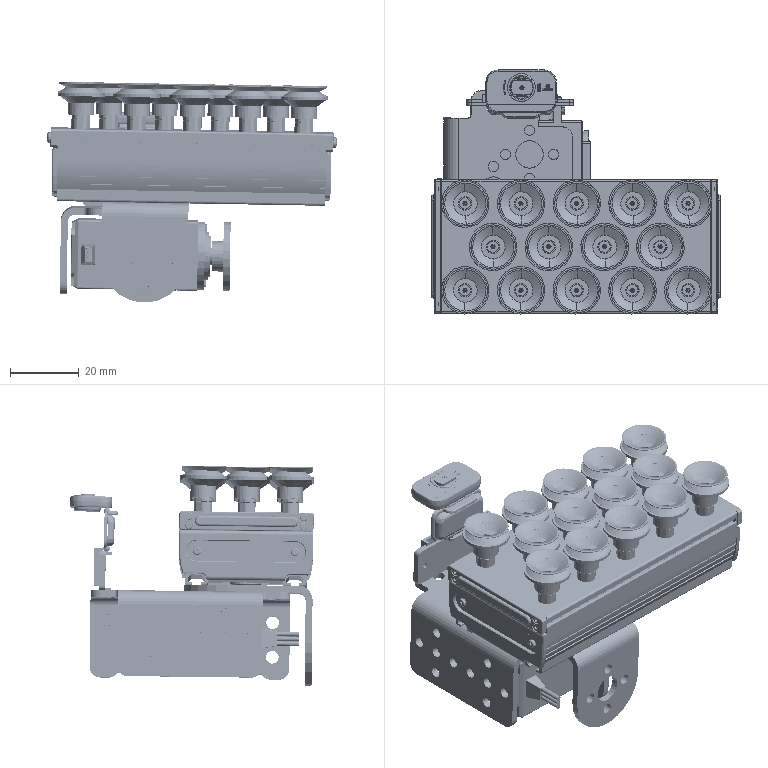Assembly | SolidWorks | mm | 78 component files | 81 solids | 4915 faces | box 84.02 x 70.93 x 64.22 mm | volume 84941 mm3 | cylinder 2079 | plane 1683 | cone 802 | spline 291 | torus 36 | sphere 24 | commonest cylinder face diameters 1.623 x328 2.074 x328 5.4 x168 1.8 x90 3 x78 5.8 x75 1.2 x74 3.3 x56
Bill of materials:
01-Profile | 1 |  | Long, constant-section, open-bottom channel-shaped profile with a flat top plate pierced by a staggered grid of holes, plus longitudinal grooves and slots along the side walls and foot features.
02-TopCoverPlate | 1 |  | Thin, flat rectangular plate with a U-shaped open slot coming in from one short end.
03-EndPlate | 2 |  | Thin plate, roughly rectangular, with a raised or recessed obround pad on one face, two small through holes, rounded edges and a stepped tab on one long edge.
04-SealingPlate | 2 |  | Long, narrow rectangular bar with chamfered corners, a long raised obround rib along one face, and two pairs of holes at the ends.
05-M4Screw | 8 |  | Socket-head screw-like shape: a cylindrical head with a hex socket and a smooth cylindrical shank with a chamfered tip.
06-M4PhillipsScrew | 4 |  | Pan- or cheese-head screw-like shape with a cross-shaped recess in the head and a smooth cylindrical shank with a chamfered tip.
07-Busbar | 1 |  | Rectangular block with chamfered corners and a stepped cylindrical spigot sticking out of one face near one end.
08-SoftRubberSuctionCup | 14 |  | Rotationally symmetric part with a cup shape: a conical inner bowl, two stacked flared lips or flanges, and a cylindrical stem with a small central through hole.
09-SuctionCupConnector | 14 |  | Fitting-like part made of a hexagonal body split by a circumferential groove, a reduced neck, and a short cylindrical spigot with a chamfered end. It has a central bore.
10-SuctionCupAirHoleScrew | 14 |  | Low, flat-headed fastener-like part: a thin wide disc head with a hex socket and a cylindrical shank with a chamfered end.
11-RetainingPlate | 2 |  | Thin, flat rectangular strip with chamfered corners and two round through holes at each end.
L Shape Bracket | 1 |  | L-shaped bent bracket of uniform thin thickness. Each leg has a rounded end and a hole pattern: one large central hole surrounded by four smaller holes.
luoding | 2 |  | Solid stepped cylinder: a long plain shaft with a shorter, larger-diameter collar or head at one end. Both end faces are flat.
Servo Bracket - universal | 1 |  | Sheet-metal-style U-shaped bracket. The flat web has a notched outline and many holes, and two legs are bent down from opposite ends. Each leg has rounded corners and two holes.
servo body | 1 |  | Compact rectangular housing, about 54 x 41 x 21 mm, with mounting holes of about 4 mm diameter, cylindrical features of about 20 mm diameter, and three separate small pin bodies about 1.4 x 1.5 x 6.5 mm.
servo dise v1 | 1 |  | Circular flange disc with a raised cylindrical hub on one face. It has a central through bore and four holes evenly spaced on a bolt circle.
TowerPro-MG995_pulley v1 | 1 |  | Cylindrical sleeve. A short section at one end has external straight teeth (spline or serration). A bore opens at the toothed end and appears to end in a conical bottom.
mecanumArm_DATAKIT_112 | 1 |  | Thin rectangular plate with rounded corners and one through hole near each end. A small tab stands up perpendicular from each long edge at mid-length. Each tab has two small holes and chamfered corners.
mecanumArm_DATAKIT_115 | 1 |  | Elongated bar-shaped body with a flat face and a rounded, convex opposite side. The ends taper and curve. A cylindrical rod or boss runs along the central part of one long edge, below the body.
mecanumArm_DATAKIT_117 | 1 |  | Very thin, narrow, curved strip shaped like a circular-arc segment, with rounded ends.
mecanumArm_DATAKIT_119 | 1 |  | Thick flat plate shaped like a circle cut by two parallel straight chords. It has a central stepped (counterbored) recess in one face.
mecanumArm_DATAKIT_121 | 1 |  | Rounded rectangular housing. The top face has a raised circular ring around a recessed disc with concentric-arc embossing. There is a grid of small dots and faint surface markings. A small cylindrical protrusion sticks out of one side, and the base is stepped and narrower.
mecanumArm_DATAKIT_123 | 1 |  | Rounded-rectangle panel or cover with a raised, rounded pad on one face. Four short cylindrical knuckle bosses sit in pairs on the two long edges. In profile it has rounded beads at the edges and a perpendicular flange near one edge.
mecanumArm_DATAKIT_125 | 1 |  | Pillow-shaped rounded-rectangle cover with one flat face and one domed face with generous edge rounds. A single cylindrical rod or knuckle runs parallel to one long edge at mid-length, offset from the body.
mecanumArm_DATAKIT_128 | 1 |  | Thin flat plate bent into a hat- or Z-joggle profile: a raised central web with a large central round hole, stepped down at each end to offset end flanges. Each flange has rounded outer corners and one small round hole. The long edges of the web have several small rectangular steps and notches.
Mates:
1. concentric | Servo Bracket - universal v1_DATAKIT_49-1/Servo Bracket - universal-1 face at (-5.311, 174.099, 12.05) dir (0.9998, 0, -0.01745) r 1.85 | Servo MG996 v1_DATAKIT_52-1/servo body-1 face at (28.584, 174.099, 11.458) dir (-0.9998, 0, 0.01745) r 2.1
2. concentric | Servo Bracket - universal v1_DATAKIT_49-1/Servo Bracket - universal-1 face at (-5.136, 173.974, 22.047) dir (0.9998, 0, -0.01745) r 1.85 | Servo MG996 v1_DATAKIT_52-1/servo body-1 face at (28.759, 173.974, 21.456) dir (-0.9998, 0, 0.01745) r 2.1
3. coincident | Servo Bracket - universal v1_DATAKIT_49-1/Servo Bracket - universal-1 face at (26.294, 174.771, 17.77) dir (0.9998, 0, -0.01745) | Servo MG996 v1_DATAKIT_52-1/servo body-1 face at (26.266, 150.038, 16.197) dir (-0.9998, 0, 0.01745)
4. concentric | Servo Bracket - universal v1_DATAKIT_49-1/Servo Bracket - universal-1 face at (19.466, 139.394, 27.684) dir (0.01745, -0.01259, 0.9998) r 4 | L Shape Bracket-1 face at (19.501, 139.369, 29.684) dir (0.01745, -0.01259, 0.9998) r 4
5. concentric | Servo Bracket - universal v1_DATAKIT_49-1/Servo Bracket - universal-1 face at (19.467, 146.394, 27.772) dir (0.01745, -0.01259, 0.9998) r 1.5 | L Shape Bracket-1 face at (19.502, 146.369, 29.772) dir (0.01745, -0.01259, 0.9998) r 1.5
6. coincident | Servo Bracket - universal v1_DATAKIT_49-1/Servo Bracket - universal-1 face at (13.504, 149.868, 29.921) dir (0.01745, -0.01259, 0.9998) | L Shape Bracket-1 face at (19.499, 133.12, 29.605) dir (-0.01745, 0.01259, -0.9998)
7. width | 02-TopCoverPlate-1 face at (273.808, -10.239, 26.969) dir (-0.03327, 0.001058, -0.9994) | 02-TopCoverPlate-1 face at (196.966, -2.76, 52.197) dir (0.03327, -0.001058, 0.9994) | 01-Profile-1 face at (197.387, -0.602, 58.564) dir (0.03327, -0.001058, 0.9994) | 01-Profile-1 face at (195.871, -4.065, 23.191) dir (-0.03327, 0.001058, -0.9994)
8. coincident | 02-TopCoverPlate-1 face at (274.561, -10.263, 49.606) dir (0.9948, -0.0962, -0.03322) | 01-Profile-1 face at (273.268, -19.732, 38.308) dir (0.9948, -0.0962, -0.03322)
9. coincident | 02-TopCoverPlate-1 face at (210.019, -4.047, 40.43) dir (-0.09618, -0.9954, 0.002148) | 01-Profile-1 face at (274.544, -10.263, 49.081) dir (0.09618, 0.9954, -0.002148)
10. concentric | 03-EndPlate-2 face at (195.401, -10.124, 26.652) dir (0.9948, -0.0962, -0.03322) r 0.75 | 01-Profile-1 face at (195.401, -10.124, 26.652) dir (-0.9948, 0.0962, 0.03322) r 0.4863
11. concentric | 03-EndPlate-2 face at (196.349, -10.154, 55.136) dir (0.9948, -0.0962, -0.03322) r 0.75 | 01-Profile-1 face at (196.349, -10.154, 55.136) dir (-0.9948, 0.0962, 0.03322) r 0.4863
12. coincident | 03-EndPlate-2 face at (195.875, -10.139, 40.894) dir (0.9948, -0.0962, -0.03322) | 01-Profile-1 face at (195.673, -12.229, 40.899) dir (-0.9948, 0.0962, 0.03322)
13. concentric | 11-RetainingPlate-2 face at (195.722, -17.472, 57.551) dir (-0.9948, 0.0962, 0.03322) r 0.645 | 01-Profile-1 face at (195.722, -17.472, 57.551) dir (-0.9948, 0.0962, 0.03322) r 0.4863
14. concentric | 11-RetainingPlate-2 face at (195.462, -20.16, 57.557) dir (-0.9948, 0.0962, 0.03322) r 0.645 | 01-Profile-1 face at (195.462, -20.16, 57.557) dir (-0.9948, 0.0962, 0.03322) r 0.4863
15. coincident | 11-RetainingPlate-2 face at (195.038, -18.798, 40.913) dir (0.9948, -0.0962, -0.03322) | 01-Profile-1 face at (195.673, -12.229, 40.899) dir (-0.9948, 0.0962, 0.03322)
16. concentric | 11-RetainingPlate-2 face at (195.722, -17.472, 57.551) dir (-0.9948, 0.0962, 0.03322) r 0.645 | 04-SealingPlate-2 face at (193.633, -17.27, 57.621) dir (-0.9948, 0.0962, 0.03322) r 1.2
17. concentric | 04-SealingPlate-2 face at (193.373, -19.958, 57.626) dir (-0.9948, 0.0962, 0.03322) r 1.2 | 01-Profile-1 face at (195.462, -20.16, 57.557) dir (-0.9948, 0.0962, 0.03322) r 0.4863
18. coincident | 11-RetainingPlate-2 face at (194.74, -18.77, 40.923) dir (-0.9948, 0.0962, 0.03322) | 04-SealingPlate-2 face at (194.74, -18.77, 40.923) dir (0.9948, -0.0962, -0.03322)
19. concentric | 07-Busbar-1 face at (210.142, -2.778, 40.427) dir (-0.09618, -0.9954, 0.002148) r 4.5 | 02-TopCoverPlate-1 face at (210.019, -4.047, 40.43) dir (0.09618, 0.9954, -0.002148) r 6.75
20. width | 07-Busbar-1 face at (199.159, -16.466, 49.183) dir (0.03327, -0.001058, 0.9994) | 07-Busbar-1 face at (252.618, -21.672, 30.589) dir (-0.03327, 0.001058, -0.9994) | 01-Profile-1 face at (194.13, -21.465, 21.429) dir (-0.03327, 0.001058, -0.9994) | 01-Profile-1 face at (196.322, -12.25, 60.388) dir (0.03327, -0.001058, 0.9994)
21. coincident | 07-Busbar-1 face at (198.879, -16.457, 40.788) dir (-0.09618, -0.9954, 0.002148) | 01-Profile-1 face at (272.434, -23.6, 24.524) dir (0.09618, 0.9954, -0.002148)
22. concentric | 06-M4PhillipsScrew-3 face at (197.789, -10.355, 26.572) dir (-0.9948, 0.0962, 0.03322) r 0.6 | 03-EndPlate-2 face at (195.401, -10.124, 26.652) dir (0.9948, -0.0962, -0.03322) r 0.75
23. coincident | 06-M4PhillipsScrew-3 face at (194.953, -10.08, 26.667) dir (0.9948, -0.0962, -0.03322) | 03-EndPlate-2 face at (194.953, -10.08, 26.667) dir (-0.9948, 0.0962, 0.03322)
24. concentric | 06-M4PhillipsScrew-4 face at (198.737, -10.385, 55.057) dir (-0.9948, 0.0962, 0.03322) r 0.6 | 03-EndPlate-2 face at (196.349, -10.154, 55.136) dir (0.9948, -0.0962, -0.03322) r 0.75
25. coincident | 06-M4PhillipsScrew-4 face at (195.902, -10.111, 55.151) dir (0.9948, -0.0962, -0.03322) | 03-EndPlate-2 face at (194.953, -10.08, 26.667) dir (-0.9948, 0.0962, 0.03322)
26. concentric | 05-M4Screw-10 face at (198.447, -20.448, 57.457) dir (-0.9948, 0.0962, 0.03322) r 0.6 | 04-SealingPlate-2 face at (193.373, -19.958, 57.626) dir (-0.9948, 0.0962, 0.03322) r 1.2
27. coincident | 05-M4Screw-10 face at (194.418, -20.059, 57.591) dir (0.9948, -0.0962, -0.03322) | 04-SealingPlate-2 face at (194.356, -20.701, 57.593) dir (-0.9948, 0.0962, 0.03322)
28. concentric | 05-M4Screw-12 face at (198.707, -17.761, 57.451) dir (-0.9948, 0.0962, 0.03322) r 0.6 | 04-SealingPlate-2 face at (193.633, -17.27, 57.621) dir (-0.9948, 0.0962, 0.03322) r 1.2
29. coincident | 05-M4Screw-12 face at (194.678, -17.371, 57.586) dir (0.9948, -0.0962, -0.03322) | 04-SealingPlate-2 face at (194.616, -18.013, 57.587) dir (-0.9948, 0.0962, 0.03322)
30. concentric | 05-M4Screw-11 face at (197.599, -17.726, 24.17) dir (-0.9948, 0.0962, 0.03322) r 0.6 | 04-SealingPlate-2 face at (192.525, -17.235, 24.339) dir (-0.9948, 0.0962, 0.03322) r 1.2
31. coincident | 05-M4Screw-11 face at (193.57, -17.336, 24.304) dir (0.9948, -0.0962, -0.03322) | 04-SealingPlate-2 face at (193.508, -17.978, 24.305) dir (-0.9948, 0.0962, 0.03322)
32. concentric | 05-M4Screw-8 face at (197.339, -20.413, 24.175) dir (-0.9948, 0.0962, 0.03322) r 0.6 | 04-SealingPlate-2 face at (192.266, -19.923, 24.345) dir (-0.9948, 0.0962, 0.03322) r 0.645
33. coincident | 05-M4Screw-8 face at (193.31, -20.024, 24.31) dir (0.9948, -0.0962, -0.03322) | 04-SealingPlate-2 face at (193.248, -20.666, 24.311) dir (-0.9948, 0.0962, 0.03322)
34. concentric | 00-VacuumSuctionCupAssembly face at (175.979, -9.357, 27.819) dir (-0.09618, -0.9954, 0.002148) r 0.9 | 00-VacuumSuctionCupAssembly face at (175.099, -18.465, 27.839) dir (0.09618, 0.9954, -0.002148) r 0.87
35. concentric | 00-VacuumSuctionCupAssembly face at (176.614, -2.788, 27.805) dir (-0.09618, -0.9954, 0.002148) r 1.459 | 00-VacuumSuctionCupAssembly face at (175.979, -9.357, 27.819) dir (-0.09618, -0.9954, 0.002148) r 0.9
36. coincident | 00-VacuumSuctionCupAssembly face at (177.189, -13.995, 27.829) dir (0.09618, 0.9954, -0.002148) | 00-VacuumSuctionCupAssembly face at (177.487, -14.024, 27.829) dir (-0.09618, -0.9954, 0.002148)
37. coincident | 00-VacuumSuctionCupAssembly face at (175.979, -9.357, 27.819) dir (-0.09618, -0.9954, 0.002148) | 00-VacuumSuctionCupAssembly face at (175.979, -9.357, 27.819) dir (0.09618, 0.9954, -0.002148)
38. concentric | 01-Profile-1 face at (200.925, -22.107, 28.106) dir (-0.09618, -0.9954, 0.002148) r 1.285 | 00-VacuumSuctionCupAssembly face at (176.614, -2.788, 27.805) dir (-0.09618, -0.9954, 0.002148) r 1.459
39. coincident | 01-Profile-1 face at (195.427, -21.507, 60.408) dir (-0.09618, -0.9954, 0.002148) | 00-VacuumSuctionCupAssembly face at (176.383, -5.177, 27.81) dir (0.09618, 0.9954, -0.002148)
40. concentric | 10-SuctionCupAirHoleScrew-35 face at (49.001, -12.826, -0.6438) dir (0, -1, 0) r 0.9 | 08-SoftRubberSuctionCup-34 face at (49.001, -21.976, -0.6438) dir (0, 1, 0) r 0.87
41. coincident | 10-SuctionCupAirHoleScrew-35 face at (50.651, -17.326, -0.6438) dir (0, 1, 0) | 08-SoftRubberSuctionCup-34 face at (50.951, -17.326, -0.6438) dir (0, -1, 0)
42. concentric | 09-SuctionCupConnector-34 face at (49.001, -6.226, -0.6438) dir (0, -1, 0) r 1.459 | 08-SoftRubberSuctionCup-34 face at (49.001, -12.826, -0.6438) dir (0, -1, 0) r 3.75
43. coincident | 09-SuctionCupConnector-34 face at (49.001, -12.826, -0.6438) dir (0, -1, 0) | 08-SoftRubberSuctionCup-34 face at (49.001, -12.826, -0.6438) dir (0, 1, 0)
44. concentric | 08-SoftRubberSuctionCup-31 face at (200.521, -26.288, 28.115) dir (-0.09618, -0.9954, 0.002148) r 3.75 | 09-SuctionCupConnector-31 face at (201.156, -19.719, 28.101) dir (-0.09618, -0.9954, 0.002148) r 1.459
45. coincident | 08-SoftRubberSuctionCup-31 face at (200.521, -26.288, 28.115) dir (0.09618, 0.9954, -0.002148) | 09-SuctionCupConnector-31 face at (200.521, -26.288, 28.115) dir (-0.09618, -0.9954, 0.002148)
46. concentric | 10-SuctionCupAirHoleScrew-32 face at (200.752, -23.899, 28.11) dir (-0.09618, -0.9954, 0.002148) r 0.9 | 08-SoftRubberSuctionCup-31 face at (200.521, -26.288, 28.115) dir (-0.09618, -0.9954, 0.002148) r 3.75
47. coincident | 10-SuctionCupAirHoleScrew-32 face at (201.962, -28.537, 28.12) dir (0.09618, 0.9954, -0.002148) | 08-SoftRubberSuctionCup-31 face at (201.185, -28.462, 28.12) dir (-0.09618, -0.9954, 0.002148)
48. concentric | 09-SuctionCupConnector-31 face at (201.156, -19.719, 28.101) dir (-0.09618, -0.9954, 0.002148) r 1.459 | 01-Profile-1 face at (200.925, -22.107, 28.106) dir (-0.09618, -0.9954, 0.002148) r 1.285
49. coincident | 09-SuctionCupConnector-31 face at (200.925, -22.107, 28.106) dir (0.09618, 0.9954, -0.002148) | 01-Profile-1 face at (195.427, -21.507, 60.408) dir (-0.09618, -0.9954, 0.002148)
50. concentric | 08-SoftRubberSuctionCup-6 face at (208.998, -27.08, 40.439) dir (-0.09618, -0.9954, 0.002148) r 3.75 | 09-SuctionCupConnector-6 face at (209.633, -20.511, 40.425) dir (-0.09618, -0.9954, 0.002148) r 1.459
51. coincident | 08-SoftRubberSuctionCup-6 face at (208.998, -27.08, 40.439) dir (0.09618, 0.9954, -0.002148) | 09-SuctionCupConnector-6 face at (208.998, -27.08, 40.439) dir (-0.09618, -0.9954, 0.002148)
52. concentric | 10-SuctionCupAirHoleScrew-12 face at (209.229, -24.692, 40.434) dir (-0.09618, -0.9954, 0.002148) r 0.9 | 09-SuctionCupConnector-6 face at (209.633, -20.511, 40.425) dir (-0.09618, -0.9954, 0.002148) r 1.459
53. coincident | 10-SuctionCupAirHoleScrew-12 edge at (208.797, -29.171, 40.444) dir (-0.09618, -0.9954, 0.002148) r 1.65 | 08-SoftRubberSuctionCup-6 face at (209.662, -29.254, 40.444) dir (-0.09618, -0.9954, 0.002148)
54. concentric | 09-SuctionCupConnector-6 face at (209.633, -20.511, 40.425) dir (-0.09618, -0.9954, 0.002148) r 1.459 | 01-Profile-1 face at (209.402, -22.9, 40.43) dir (-0.09618, -0.9954, 0.002148) r 1.285
55. coincident | 09-SuctionCupConnector-6 face at (209.402, -22.9, 40.43) dir (0.09618, 0.9954, -0.002148) | 01-Profile-1 face at (195.427, -21.507, 60.408) dir (-0.09618, -0.9954, 0.002148)
56. concentric | mecanumArm_DATAKIT_123-1 face at (-8.853, 4.135, 24.626) dir (1, 0, 0) r 0.9 | mecanumArm_DATAKIT_125-1 face at (-7.293, 4.135, 24.626) dir (1, 0, 0) r 0.975
57. coincident | mecanumArm_DATAKIT_123-1 face at (-0.0928, 4.135, 24.626) dir (-1, 0, 0) | mecanumArm_DATAKIT_125-1 face at (-0.0928, 4.135, 24.626) dir (1, 0, 0)
58. concentric | mecanumArm_DATAKIT_115-1 face at (-0.07848, 4.232, 13.826) dir (-1, 0, 0) r 0.975 | mecanumArm_DATAKIT_123-1 face at (-8.853, 4.232, 13.826) dir (1, 0, 0) r 0.9
59. concentric | mecanumArm_DATAKIT_115-1 edge at (-3.678, 4.915, 11.276) dir (0, 1, 0) r 0.6 | mecanumArm_DATAKIT_121-1 face at (-3.678, 4.741, 11.276) dir (0, 1, 0) r 0.6
60. coincident | mecanumArm_DATAKIT_115-1 face at (5.791, 5.218, 10.301) dir (0, 1, 0) | mecanumArm_DATAKIT_121-1 face at (5.787, 5.218, 10.264) dir (0, -1, 0)
61. coincident | mecanumArm_DATAKIT_119-1 face at (-3.875, 9.957, 9.852) dir (0.00391, 0, 1) | mecanumArm_DATAKIT_121-1 face at (-3.684, 10.021, 9.851) dir (-0.00391, 0, -1)
62. coincident | mecanumArm_DATAKIT_117-1 face at (-1.404, 10.925, 9.722) dir (0.00391, 0, 1) | mecanumArm_DATAKIT_121-1 face at (-1.379, 10.951, 9.722) dir (-0.00391, 0, -1)
63. concentric | mecanumArm_DATAKIT_112-1 face at (8.748, 5.196, 31.263) dir (0, -0.9999, -0.01188) r 0.75 | mecanumArm_DATAKIT_128-1 face at (8.748, 5.196, 31.263) dir (0, 0.9999, 0.01188) r 0.75
64. coincident | mecanumArm_DATAKIT_112-1 face at (-3.642, 5.196, 31.282) dir (0, 0.9999, 0.01188) | mecanumArm_DATAKIT_128-1 face at (6.314, 5.148, 35.343) dir (0, -0.9999, -0.01188)